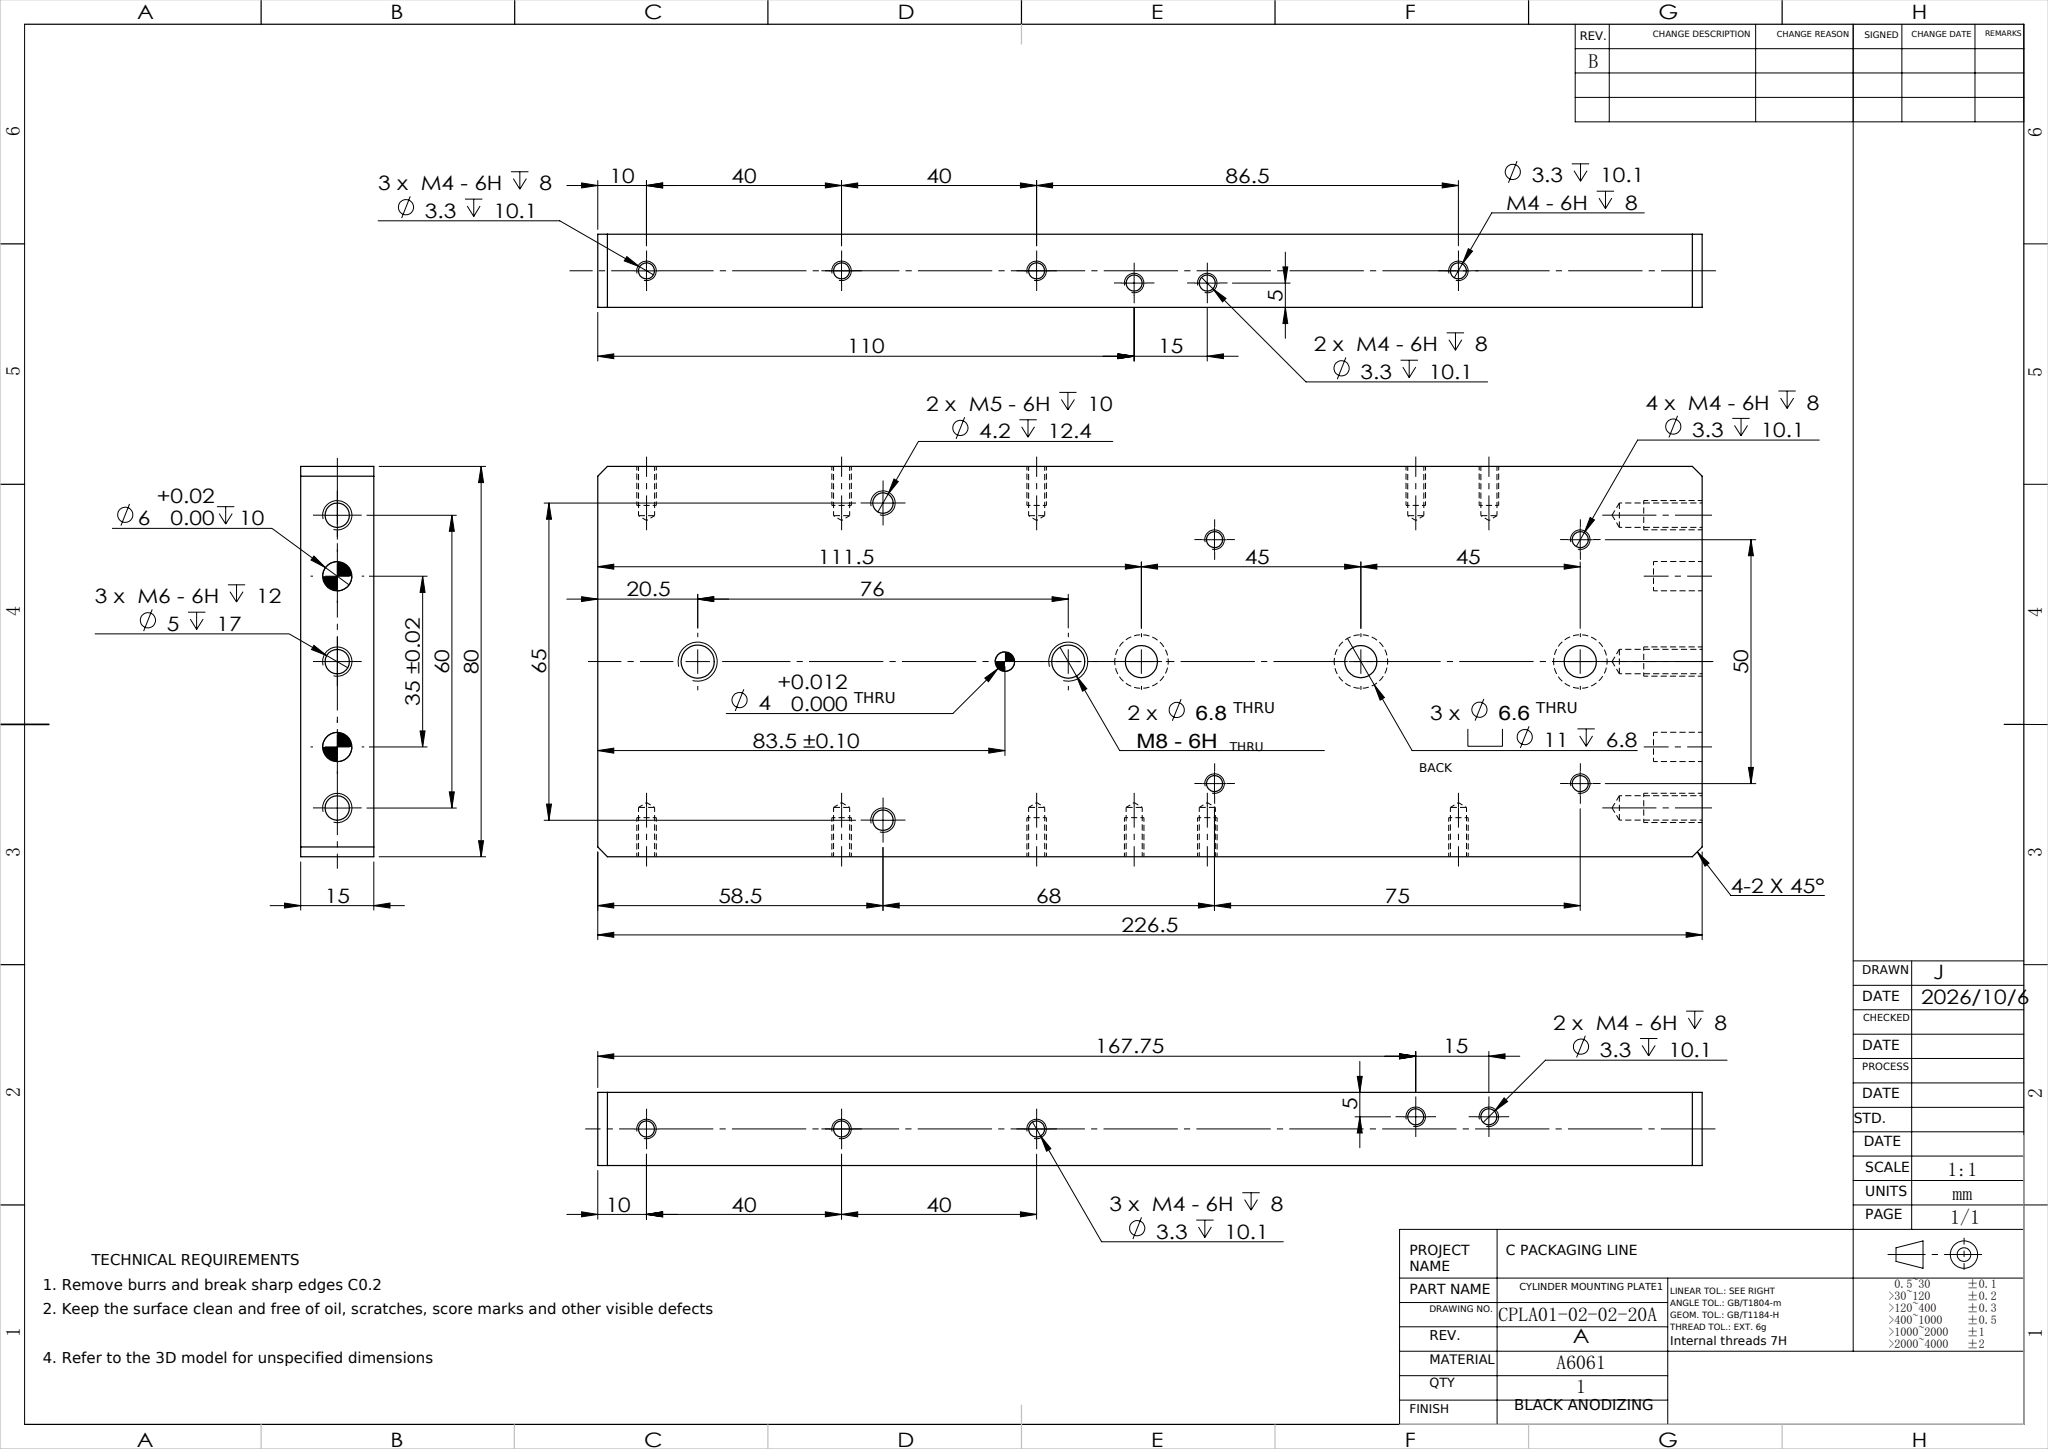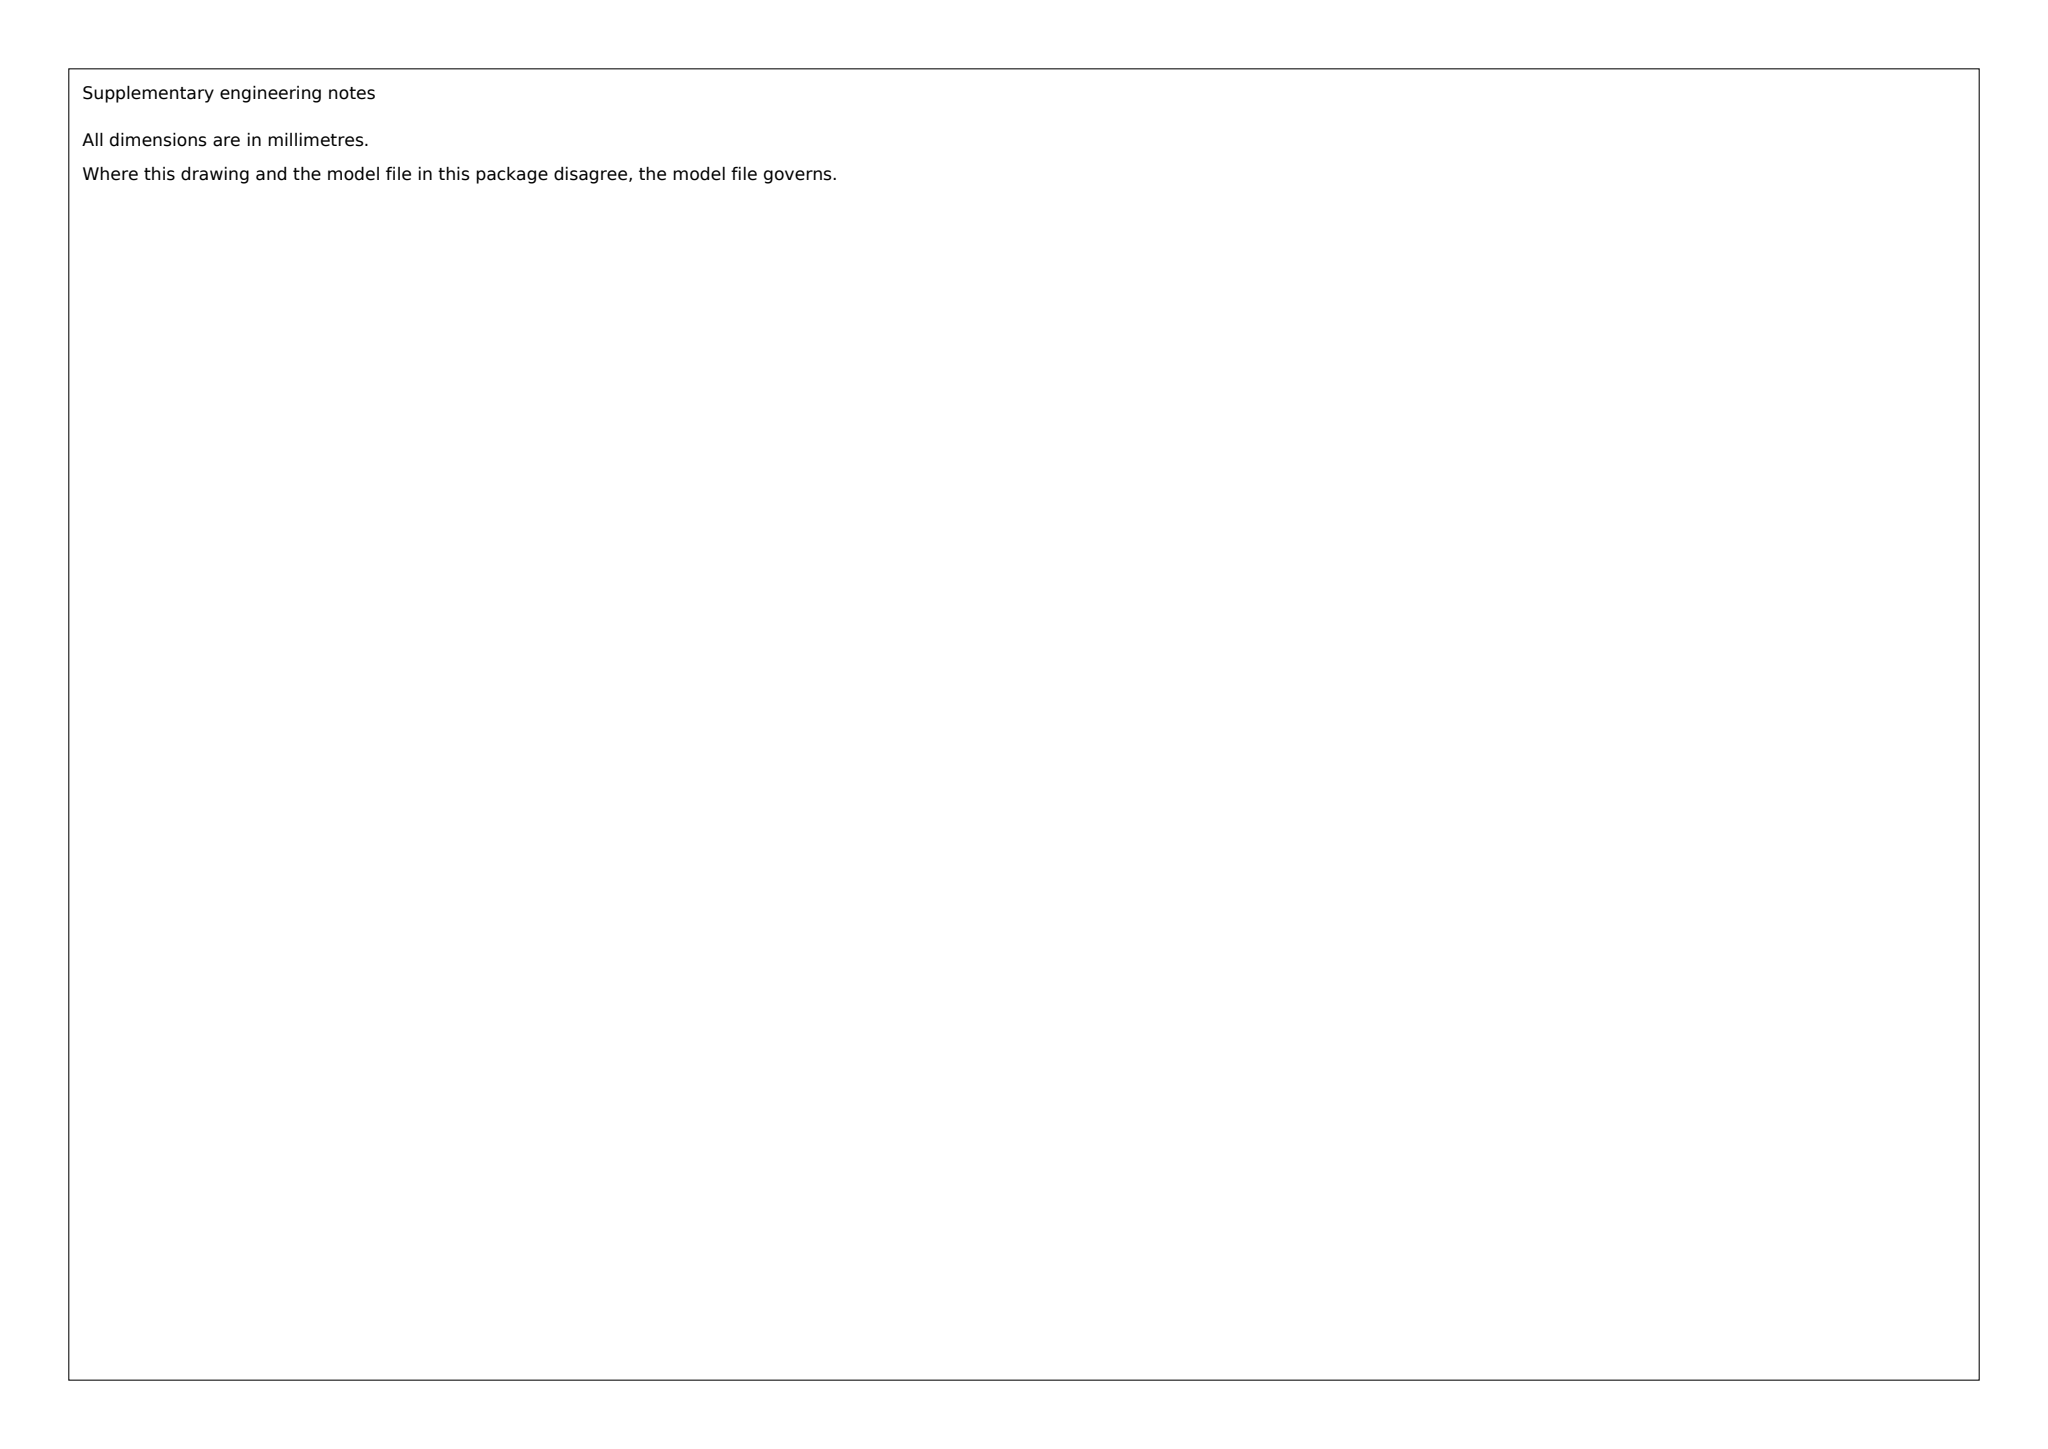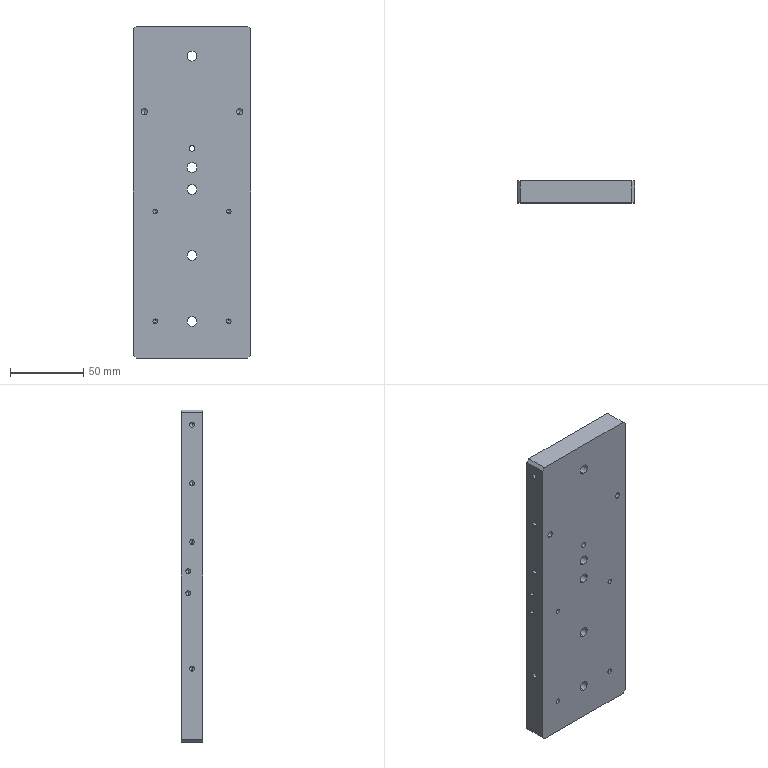Part | SolidWorks | mm | 1 solid | 117 faces | box 80 x 15 x 226.5 mm | volume 264332 mm3 | cylinder 62 | cone 40 | plane 15 | commonest cylinder face diameters 3.3 x30 11 x6 6.6 x6 5 x6 4.2 x4 6.8 x4 6 x4 4 x2